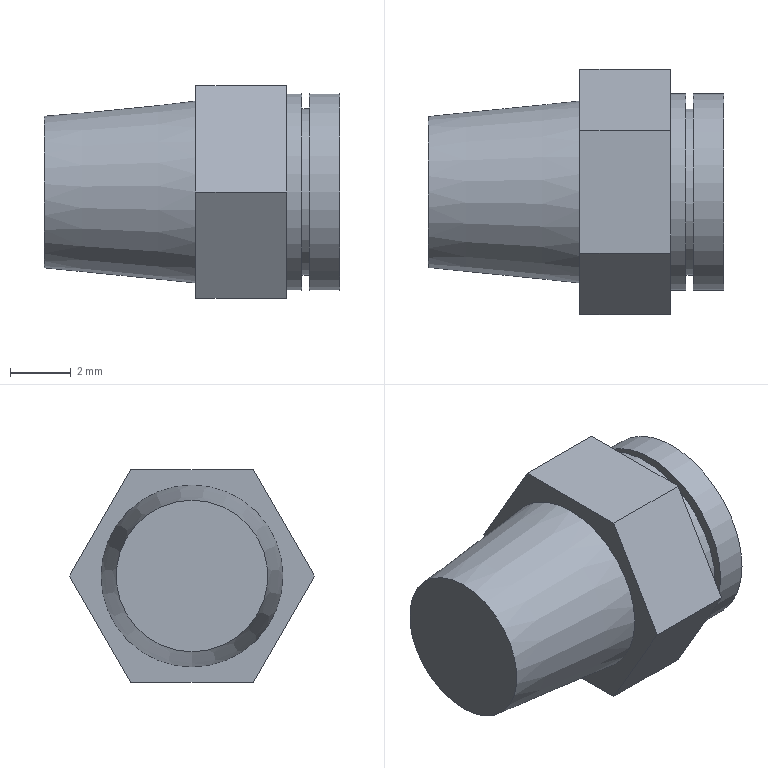Component | NX | AIR_HOSE_CONN_2 | 1 solid | 18 faces | box 9.75 x 8.08 x 7 mm | volume 175 mm3 | plane 13 | cylinder 4 | cone 1 | commonest cylinder face diameters 6.5 x2 5.5 x1 5 x1
STEP:
#1=CARTESIAN_POINT('',(0.,0.,0.));
#2=DIRECTION('',(0.,0.,1.));
#3=DIRECTION('',(1.,0.,0.));
#4=AXIS2_PLACEMENT_3D('',#1,#2,#3);
#5=CARTESIAN_POINT('',(51.,-7.,-6.5));
#6=VERTEX_POINT('',#5);
#7=CARTESIAN_POINT('',(51.,-7.,-4.));
#8=DIRECTION('',(-1.,0.,0.));
#9=DIRECTION('',(0.,0.,-1.));
#10=AXIS2_PLACEMENT_3D('',#7,#8,#9);
#11=CIRCLE('',#10,2.5);
#12=CARTESIAN_POINT('',(56.,-7.,-4.));
#13=DIRECTION('',(1.,0.,0.));
#14=DIRECTION('',(0.,0.,1.));
#15=AXIS2_PLACEMENT_3D('',#12,#13,#14);
#16=CONICAL_SURFACE('',#15,3.,0.09967);
#17=CARTESIAN_POINT('',(9.425,-5.));
#18=DIRECTION('',(-1.,0.));
#19=VECTOR('',#18,1.);
#20=LINE('',#17,#19);
#21=(GEOMETRIC_REPRESENTATION_CONTEXT(2)PARAMETRIC_REPRESENTATION_CONTEXT()REPRESENTATION_CONTEXT('',''));
#22=DEFINITIONAL_REPRESENTATION('',(#20),#21);
#23=PCURVE('',#16,#22);
#24=CARTESIAN_POINT('',(51.,-7.,-1.5));
#25=DIRECTION('',(1.,0.,0.));
#26=DIRECTION('',(0.,0.,1.));
#27=AXIS2_PLACEMENT_3D('',#24,#25,#26);
#28=PLANE('',#27);
#29=CARTESIAN_POINT('',(-5.,0.));
#30=CARTESIAN_POINT('',(-5.,4.33));
#31=CARTESIAN_POINT('',(-1.25,2.165));
#32=CARTESIAN_POINT('',(2.5,0.));
#33=CARTESIAN_POINT('',(-1.25,-2.165));
#34=CARTESIAN_POINT('',(-5.,-4.33));
#35=CARTESIAN_POINT('',(-5.,0.));
#36=(BOUNDED_CURVE()B_SPLINE_CURVE(2,(#29,#30,#31,#32,#33,#34,#35),.UNSPECIFIED.,.T.,.F.)B_SPLINE_CURVE_WITH_KNOTS((1,2,2,2,2,1),(-2.094,0.,2.094,4.189,6.283,8.378),.UNSPECIFIED.)CURVE()GEOMETRIC_REPRESENTATION_ITEM()RATIONAL_B_SPLINE_CURVE((1.,0.5,1.,0.5,1.,0.5,1.))REPRESENTATION_ITEM(''));
#37=(GEOMETRIC_REPRESENTATION_CONTEXT(2)PARAMETRIC_REPRESENTATION_CONTEXT()REPRESENTATION_CONTEXT('',''));
#38=DEFINITIONAL_REPRESENTATION('',(#36),#37);
#39=PCURVE('',#28,#38);
#40=SURFACE_CURVE('',#11,(#23,#39),.PCURVE_S1.);
#41=EDGE_CURVE('',#6,#6,#40,.T.);
#42=ORIENTED_EDGE('',*,*,#41,.F.);
#43=CARTESIAN_POINT('',(56.,-7.,-7.));
#44=VERTEX_POINT('',#43);
#45=CARTESIAN_POINT('',(51.,-7.,-6.5));
#46=CARTESIAN_POINT('',(56.,-7.,-7.));
#47=B_SPLINE_CURVE_WITH_KNOTS('',1,(#45,#46),.UNSPECIFIED.,.F.,.F.,(2,2),(-5.025,0.),.PIECEWISE_BEZIER_KNOTS.);
#48=CARTESIAN_POINT('',(9.425,0.));
#49=DIRECTION('',(0.,1.));
#50=VECTOR('',#49,1.);
#51=LINE('',#48,#50);
#52=(GEOMETRIC_REPRESENTATION_CONTEXT(2)PARAMETRIC_REPRESENTATION_CONTEXT()REPRESENTATION_CONTEXT('',''));
#53=DEFINITIONAL_REPRESENTATION('',(#51),#52);
#54=PCURVE('',#16,#53);
#55=CARTESIAN_POINT('',(3.142,0.));
#56=DIRECTION('',(0.,1.));
#57=VECTOR('',#56,1.);
#58=LINE('',#55,#57);
#59=(GEOMETRIC_REPRESENTATION_CONTEXT(2)PARAMETRIC_REPRESENTATION_CONTEXT()REPRESENTATION_CONTEXT('',''));
#60=DEFINITIONAL_REPRESENTATION('',(#58),#59);
#61=PCURVE('',#16,#60);
#62=SEAM_CURVE('',#47,(#54,#61),.PCURVE_S1.);
#63=EDGE_CURVE('',#6,#44,#62,.T.);
#64=ORIENTED_EDGE('',*,*,#63,.T.);
#65=CARTESIAN_POINT('',(56.,-7.,-4.));
#66=DIRECTION('',(-1.,0.,0.));
#67=DIRECTION('',(0.,0.,-1.));
#68=AXIS2_PLACEMENT_3D('',#65,#66,#67);
#69=CIRCLE('',#68,3.);
#70=CARTESIAN_POINT('',(9.425,0.));
#71=DIRECTION('',(-1.,0.));
#72=VECTOR('',#71,1.);
#73=LINE('',#70,#72);
#74=(GEOMETRIC_REPRESENTATION_CONTEXT(2)PARAMETRIC_REPRESENTATION_CONTEXT()REPRESENTATION_CONTEXT('',''));
#75=DEFINITIONAL_REPRESENTATION('',(#73),#74);
#76=PCURVE('',#16,#75);
#77=CARTESIAN_POINT('',(56.,-7.,-4.));
#78=DIRECTION('',(-1.,0.,0.));
#79=DIRECTION('',(0.,0.,-1.));
#80=AXIS2_PLACEMENT_3D('',#77,#78,#79);
#81=PLANE('',#80);
#82=CARTESIAN_POINT('',(0.,0.));
#83=DIRECTION('',(1.,0.));
#84=AXIS2_PLACEMENT_2D('',#82,#83);
#85=CIRCLE('',#84,3.);
#86=(GEOMETRIC_REPRESENTATION_CONTEXT(2)PARAMETRIC_REPRESENTATION_CONTEXT()REPRESENTATION_CONTEXT('',''));
#87=DEFINITIONAL_REPRESENTATION('',(#85),#86);
#88=PCURVE('',#81,#87);
#89=SURFACE_CURVE('',#69,(#76,#88),.PCURVE_S1.);
#90=EDGE_CURVE('',#44,#44,#89,.T.);
#91=ORIENTED_EDGE('',*,*,#90,.T.);
#92=ORIENTED_EDGE('',*,*,#63,.F.);
#93=EDGE_LOOP('',(#42,#64,#91,#92));
#94=FACE_BOUND('',#93,.T.);
#95=ADVANCED_FACE('',(#94),#16,.T.);
#96=ORIENTED_EDGE('',*,*,#41,.T.);
#97=EDGE_LOOP('',(#96));
#98=FACE_BOUND('',#97,.T.);
#99=ADVANCED_FACE('',(#98),#28,.F.);
#100=CARTESIAN_POINT('',(56.,-4.979,-7.5));
#101=VERTEX_POINT('',#100);
#102=CARTESIAN_POINT('',(56.,-9.021,-7.5));
#103=VERTEX_POINT('',#102);
#104=CARTESIAN_POINT('',(56.,-4.979,-7.5));
#105=DIRECTION('',(0.,-1.,0.));
#106=VECTOR('',#105,1.);
#107=LINE('',#104,#106);
#108=CARTESIAN_POINT('',(59.,-4.979,-7.5));
#109=DIRECTION('',(0.,-0.,-1.));
#110=DIRECTION('',(0.,1.,-0.));
#111=AXIS2_PLACEMENT_3D('',#108,#109,#110);
#112=PLANE('',#111);
#113=CARTESIAN_POINT('',(0.,-3.));
#114=DIRECTION('',(-1.,0.));
#115=VECTOR('',#114,1.);
#116=LINE('',#113,#115);
#117=(GEOMETRIC_REPRESENTATION_CONTEXT(2)PARAMETRIC_REPRESENTATION_CONTEXT()REPRESENTATION_CONTEXT('',''));
#118=DEFINITIONAL_REPRESENTATION('',(#116),#117);
#119=PCURVE('',#112,#118);
#120=CARTESIAN_POINT('',(3.5,-2.021));
#121=DIRECTION('',(-0.,1.));
#122=VECTOR('',#121,1.);
#123=LINE('',#120,#122);
#124=(GEOMETRIC_REPRESENTATION_CONTEXT(2)PARAMETRIC_REPRESENTATION_CONTEXT()REPRESENTATION_CONTEXT('',''));
#125=DEFINITIONAL_REPRESENTATION('',(#123),#124);
#126=PCURVE('',#81,#125);
#127=SURFACE_CURVE('',#107,(#119,#126),.PCURVE_S1.);
#128=EDGE_CURVE('',#101,#103,#127,.T.);
#129=ORIENTED_EDGE('',*,*,#128,.F.);
#130=CARTESIAN_POINT('',(59.,-4.979,-7.5));
#131=VERTEX_POINT('',#130);
#132=CARTESIAN_POINT('',(59.,-4.979,-7.5));
#133=DIRECTION('',(-1.,0.,0.));
#134=VECTOR('',#133,1.);
#135=LINE('',#132,#134);
#136=CARTESIAN_POINT('',(0.,0.));
#137=DIRECTION('',(0.,-1.));
#138=VECTOR('',#137,1.);
#139=LINE('',#136,#138);
#140=(GEOMETRIC_REPRESENTATION_CONTEXT(2)PARAMETRIC_REPRESENTATION_CONTEXT()REPRESENTATION_CONTEXT('',''));
#141=DEFINITIONAL_REPRESENTATION('',(#139),#140);
#142=PCURVE('',#112,#141);
#143=CARTESIAN_POINT('',(59.,-2.959,-4.));
#144=DIRECTION('',(0.,0.866,-0.5));
#145=DIRECTION('',(0.,0.5,0.866));
#146=AXIS2_PLACEMENT_3D('',#143,#144,#145);
#147=PLANE('',#146);
#148=CARTESIAN_POINT('',(-4.041,0.));
#149=DIRECTION('',(0.,-1.));
#150=VECTOR('',#149,1.);
#151=LINE('',#148,#150);
#152=(GEOMETRIC_REPRESENTATION_CONTEXT(2)PARAMETRIC_REPRESENTATION_CONTEXT()REPRESENTATION_CONTEXT('',''));
#153=DEFINITIONAL_REPRESENTATION('',(#151),#152);
#154=PCURVE('',#147,#153);
#155=SURFACE_CURVE('',#135,(#142,#154),.PCURVE_S1.);
#156=EDGE_CURVE('',#131,#101,#155,.T.);
#157=ORIENTED_EDGE('',*,*,#156,.F.);
#158=CARTESIAN_POINT('',(59.,-9.021,-7.5));
#159=VERTEX_POINT('',#158);
#160=CARTESIAN_POINT('',(59.,-4.979,-7.5));
#161=DIRECTION('',(0.,-1.,0.));
#162=VECTOR('',#161,1.);
#163=LINE('',#160,#162);
#164=CARTESIAN_POINT('',(0.,0.));
#165=DIRECTION('',(-1.,0.));
#166=VECTOR('',#165,1.);
#167=LINE('',#164,#166);
#168=(GEOMETRIC_REPRESENTATION_CONTEXT(2)PARAMETRIC_REPRESENTATION_CONTEXT()REPRESENTATION_CONTEXT('',''));
#169=DEFINITIONAL_REPRESENTATION('',(#167),#168);
#170=PCURVE('',#112,#169);
#171=CARTESIAN_POINT('',(59.,-7.,-4.));
#172=DIRECTION('',(-1.,0.,0.));
#173=DIRECTION('',(0.,0.,-1.));
#174=AXIS2_PLACEMENT_3D('',#171,#172,#173);
#175=PLANE('',#174);
#176=CARTESIAN_POINT('',(3.5,-2.021));
#177=DIRECTION('',(-0.,1.));
#178=VECTOR('',#177,1.);
#179=LINE('',#176,#178);
#180=(GEOMETRIC_REPRESENTATION_CONTEXT(2)PARAMETRIC_REPRESENTATION_CONTEXT()REPRESENTATION_CONTEXT('',''));
#181=DEFINITIONAL_REPRESENTATION('',(#179),#180);
#182=PCURVE('',#175,#181);
#183=SURFACE_CURVE('',#163,(#170,#182),.PCURVE_S1.);
#184=EDGE_CURVE('',#131,#159,#183,.T.);
#185=ORIENTED_EDGE('',*,*,#184,.T.);
#186=CARTESIAN_POINT('',(59.,-9.021,-7.5));
#187=DIRECTION('',(-1.,0.,0.));
#188=VECTOR('',#187,1.);
#189=LINE('',#186,#188);
#190=CARTESIAN_POINT('',(-4.041,0.));
#191=DIRECTION('',(0.,-1.));
#192=VECTOR('',#191,1.);
#193=LINE('',#190,#192);
#194=(GEOMETRIC_REPRESENTATION_CONTEXT(2)PARAMETRIC_REPRESENTATION_CONTEXT()REPRESENTATION_CONTEXT('',''));
#195=DEFINITIONAL_REPRESENTATION('',(#193),#194);
#196=PCURVE('',#112,#195);
#197=CARTESIAN_POINT('',(59.,-9.021,-7.5));
#198=DIRECTION('',(0.,-0.866,-0.5));
#199=DIRECTION('',(0.,0.5,-0.866));
#200=AXIS2_PLACEMENT_3D('',#197,#198,#199);
#201=PLANE('',#200);
#202=CARTESIAN_POINT('',(0.,0.));
#203=DIRECTION('',(0.,-1.));
#204=VECTOR('',#203,1.);
#205=LINE('',#202,#204);
#206=(GEOMETRIC_REPRESENTATION_CONTEXT(2)PARAMETRIC_REPRESENTATION_CONTEXT()REPRESENTATION_CONTEXT('',''));
#207=DEFINITIONAL_REPRESENTATION('',(#205),#206);
#208=PCURVE('',#201,#207);
#209=SURFACE_CURVE('',#189,(#196,#208),.PCURVE_S1.);
#210=EDGE_CURVE('',#159,#103,#209,.T.);
#211=ORIENTED_EDGE('',*,*,#210,.T.);
#212=EDGE_LOOP('',(#129,#157,#185,#211));
#213=FACE_BOUND('',#212,.T.);
#214=ADVANCED_FACE('',(#213),#112,.T.);
#215=CARTESIAN_POINT('',(56.,-11.041,-4.));
#216=VERTEX_POINT('',#215);
#217=CARTESIAN_POINT('',(56.,-9.021,-7.5));
#218=DIRECTION('',(0.,-0.5,0.866));
#219=VECTOR('',#218,1.);
#220=LINE('',#217,#219);
#221=CARTESIAN_POINT('',(0.,-3.));
#222=DIRECTION('',(-1.,0.));
#223=VECTOR('',#222,1.);
#224=LINE('',#221,#223);
#225=(GEOMETRIC_REPRESENTATION_CONTEXT(2)PARAMETRIC_REPRESENTATION_CONTEXT()REPRESENTATION_CONTEXT('',''));
#226=DEFINITIONAL_REPRESENTATION('',(#224),#225);
#227=PCURVE('',#201,#226);
#228=CARTESIAN_POINT('',(3.5,2.021));
#229=DIRECTION('',(-0.866,0.5));
#230=VECTOR('',#229,1.);
#231=LINE('',#228,#230);
#232=(GEOMETRIC_REPRESENTATION_CONTEXT(2)PARAMETRIC_REPRESENTATION_CONTEXT()REPRESENTATION_CONTEXT('',''));
#233=DEFINITIONAL_REPRESENTATION('',(#231),#232);
#234=PCURVE('',#81,#233);
#235=SURFACE_CURVE('',#220,(#227,#234),.PCURVE_S1.);
#236=EDGE_CURVE('',#103,#216,#235,.T.);
#237=ORIENTED_EDGE('',*,*,#236,.F.);
#238=ORIENTED_EDGE('',*,*,#210,.F.);
#239=CARTESIAN_POINT('',(59.,-11.041,-4.));
#240=VERTEX_POINT('',#239);
#241=CARTESIAN_POINT('',(59.,-9.021,-7.5));
#242=DIRECTION('',(0.,-0.5,0.866));
#243=VECTOR('',#242,1.);
#244=LINE('',#241,#243);
#245=CARTESIAN_POINT('',(0.,0.));
#246=DIRECTION('',(-1.,0.));
#247=VECTOR('',#246,1.);
#248=LINE('',#245,#247);
#249=(GEOMETRIC_REPRESENTATION_CONTEXT(2)PARAMETRIC_REPRESENTATION_CONTEXT()REPRESENTATION_CONTEXT('',''));
#250=DEFINITIONAL_REPRESENTATION('',(#248),#249);
#251=PCURVE('',#201,#250);
#252=CARTESIAN_POINT('',(3.5,2.021));
#253=DIRECTION('',(-0.866,0.5));
#254=VECTOR('',#253,1.);
#255=LINE('',#252,#254);
#256=(GEOMETRIC_REPRESENTATION_CONTEXT(2)PARAMETRIC_REPRESENTATION_CONTEXT()REPRESENTATION_CONTEXT('',''));
#257=DEFINITIONAL_REPRESENTATION('',(#255),#256);
#258=PCURVE('',#175,#257);
#259=SURFACE_CURVE('',#244,(#251,#258),.PCURVE_S1.);
#260=EDGE_CURVE('',#159,#240,#259,.T.);
#261=ORIENTED_EDGE('',*,*,#260,.T.);
#262=CARTESIAN_POINT('',(59.,-11.041,-4.));
#263=DIRECTION('',(-1.,0.,0.));
#264=VECTOR('',#263,1.);
#265=LINE('',#262,#264);
#266=CARTESIAN_POINT('',(-4.041,0.));
#267=DIRECTION('',(0.,-1.));
#268=VECTOR('',#267,1.);
#269=LINE('',#266,#268);
#270=(GEOMETRIC_REPRESENTATION_CONTEXT(2)PARAMETRIC_REPRESENTATION_CONTEXT()REPRESENTATION_CONTEXT('',''));
#271=DEFINITIONAL_REPRESENTATION('',(#269),#270);
#272=PCURVE('',#201,#271);
#273=CARTESIAN_POINT('',(59.,-11.041,-4.));
#274=DIRECTION('',(0.,-0.866,0.5));
#275=DIRECTION('',(0.,-0.5,-0.866));
#276=AXIS2_PLACEMENT_3D('',#273,#274,#275);
#277=PLANE('',#276);
#278=CARTESIAN_POINT('',(0.,0.));
#279=DIRECTION('',(0.,-1.));
#280=VECTOR('',#279,1.);
#281=LINE('',#278,#280);
#282=(GEOMETRIC_REPRESENTATION_CONTEXT(2)PARAMETRIC_REPRESENTATION_CONTEXT()REPRESENTATION_CONTEXT('',''));
#283=DEFINITIONAL_REPRESENTATION('',(#281),#282);
#284=PCURVE('',#277,#283);
#285=SURFACE_CURVE('',#265,(#272,#284),.PCURVE_S1.);
#286=EDGE_CURVE('',#240,#216,#285,.T.);
#287=ORIENTED_EDGE('',*,*,#286,.T.);
#288=EDGE_LOOP('',(#237,#238,#261,#287));
#289=FACE_BOUND('',#288,.T.);
#290=ADVANCED_FACE('',(#289),#201,.T.);
#291=CARTESIAN_POINT('',(56.,-9.021,-0.5));
#292=VERTEX_POINT('',#291);
#293=CARTESIAN_POINT('',(56.,-11.041,-4.));
#294=DIRECTION('',(0.,0.5,0.866));
#295=VECTOR('',#294,1.);
#296=LINE('',#293,#295);
#297=CARTESIAN_POINT('',(0.,-3.));
#298=DIRECTION('',(-1.,0.));
#299=VECTOR('',#298,1.);
#300=LINE('',#297,#299);
#301=(GEOMETRIC_REPRESENTATION_CONTEXT(2)PARAMETRIC_REPRESENTATION_CONTEXT()REPRESENTATION_CONTEXT('',''));
#302=DEFINITIONAL_REPRESENTATION('',(#300),#301);
#303=PCURVE('',#277,#302);
#304=CARTESIAN_POINT('',(-0.,4.041));
#305=DIRECTION('',(-0.866,-0.5));
#306=VECTOR('',#305,1.);
#307=LINE('',#304,#306);
#308=(GEOMETRIC_REPRESENTATION_CONTEXT(2)PARAMETRIC_REPRESENTATION_CONTEXT()REPRESENTATION_CONTEXT('',''));
#309=DEFINITIONAL_REPRESENTATION('',(#307),#308);
#310=PCURVE('',#81,#309);
#311=SURFACE_CURVE('',#296,(#303,#310),.PCURVE_S1.);
#312=EDGE_CURVE('',#216,#292,#311,.T.);
#313=ORIENTED_EDGE('',*,*,#312,.F.);
#314=ORIENTED_EDGE('',*,*,#286,.F.);
#315=CARTESIAN_POINT('',(59.,-9.021,-0.5));
#316=VERTEX_POINT('',#315);
#317=CARTESIAN_POINT('',(59.,-11.041,-4.));
#318=DIRECTION('',(0.,0.5,0.866));
#319=VECTOR('',#318,1.);
#320=LINE('',#317,#319);
#321=CARTESIAN_POINT('',(0.,0.));
#322=DIRECTION('',(-1.,0.));
#323=VECTOR('',#322,1.);
#324=LINE('',#321,#323);
#325=(GEOMETRIC_REPRESENTATION_CONTEXT(2)PARAMETRIC_REPRESENTATION_CONTEXT()REPRESENTATION_CONTEXT('',''));
#326=DEFINITIONAL_REPRESENTATION('',(#324),#325);
#327=PCURVE('',#277,#326);
#328=CARTESIAN_POINT('',(-0.,4.041));
#329=DIRECTION('',(-0.866,-0.5));
#330=VECTOR('',#329,1.);
#331=LINE('',#328,#330);
#332=(GEOMETRIC_REPRESENTATION_CONTEXT(2)PARAMETRIC_REPRESENTATION_CONTEXT()REPRESENTATION_CONTEXT('',''));
#333=DEFINITIONAL_REPRESENTATION('',(#331),#332);
#334=PCURVE('',#175,#333);
#335=SURFACE_CURVE('',#320,(#327,#334),.PCURVE_S1.);
#336=EDGE_CURVE('',#240,#316,#335,.T.);
#337=ORIENTED_EDGE('',*,*,#336,.T.);
#338=CARTESIAN_POINT('',(59.,-9.021,-0.5));
#339=DIRECTION('',(-1.,0.,0.));
#340=VECTOR('',#339,1.);
#341=LINE('',#338,#340);
#342=CARTESIAN_POINT('',(-4.041,0.));
#343=DIRECTION('',(0.,-1.));
#344=VECTOR('',#343,1.);
#345=LINE('',#342,#344);
#346=(GEOMETRIC_REPRESENTATION_CONTEXT(2)PARAMETRIC_REPRESENTATION_CONTEXT()REPRESENTATION_CONTEXT('',''));
#347=DEFINITIONAL_REPRESENTATION('',(#345),#346);
#348=PCURVE('',#277,#347);
#349=CARTESIAN_POINT('',(59.,-9.021,-0.5));
#350=DIRECTION('',(0.,0.,1.));
#351=DIRECTION('',(0.,-1.,0.));
#352=AXIS2_PLACEMENT_3D('',#349,#350,#351);
#353=PLANE('',#352);
#354=CARTESIAN_POINT('',(0.,0.));
#355=DIRECTION('',(0.,-1.));
#356=VECTOR('',#355,1.);
#357=LINE('',#354,#356);
#358=(GEOMETRIC_REPRESENTATION_CONTEXT(2)PARAMETRIC_REPRESENTATION_CONTEXT()REPRESENTATION_CONTEXT('',''));
#359=DEFINITIONAL_REPRESENTATION('',(#357),#358);
#360=PCURVE('',#353,#359);
#361=SURFACE_CURVE('',#341,(#348,#360),.PCURVE_S1.);
#362=EDGE_CURVE('',#316,#292,#361,.T.);
#363=ORIENTED_EDGE('',*,*,#362,.T.);
#364=EDGE_LOOP('',(#313,#314,#337,#363));
#365=FACE_BOUND('',#364,.T.);
#366=ADVANCED_FACE('',(#365),#277,.T.);
#367=CARTESIAN_POINT('',(56.,-4.979,-0.5));
#368=VERTEX_POINT('',#367);
#369=CARTESIAN_POINT('',(56.,-9.021,-0.5));
#370=DIRECTION('',(0.,1.,-0.));
#371=VECTOR('',#370,1.);
#372=LINE('',#369,#371);
#373=CARTESIAN_POINT('',(0.,-3.));
#374=DIRECTION('',(-1.,0.));
#375=VECTOR('',#374,1.);
#376=LINE('',#373,#375);
#377=(GEOMETRIC_REPRESENTATION_CONTEXT(2)PARAMETRIC_REPRESENTATION_CONTEXT()REPRESENTATION_CONTEXT('',''));
#378=DEFINITIONAL_REPRESENTATION('',(#376),#377);
#379=PCURVE('',#353,#378);
#380=CARTESIAN_POINT('',(-3.5,2.021));
#381=DIRECTION('',(0.,-1.));
#382=VECTOR('',#381,1.);
#383=LINE('',#380,#382);
#384=(GEOMETRIC_REPRESENTATION_CONTEXT(2)PARAMETRIC_REPRESENTATION_CONTEXT()REPRESENTATION_CONTEXT('',''));
#385=DEFINITIONAL_REPRESENTATION('',(#383),#384);
#386=PCURVE('',#81,#385);
#387=SURFACE_CURVE('',#372,(#379,#386),.PCURVE_S1.);
#388=EDGE_CURVE('',#292,#368,#387,.T.);
#389=ORIENTED_EDGE('',*,*,#388,.F.);
#390=ORIENTED_EDGE('',*,*,#362,.F.);
#391=CARTESIAN_POINT('',(59.,-4.979,-0.5));
#392=VERTEX_POINT('',#391);
#393=CARTESIAN_POINT('',(59.,-9.021,-0.5));
#394=DIRECTION('',(0.,1.,-0.));
#395=VECTOR('',#394,1.);
#396=LINE('',#393,#395);
#397=CARTESIAN_POINT('',(0.,0.));
#398=DIRECTION('',(-1.,0.));
#399=VECTOR('',#398,1.);
#400=LINE('',#397,#399);
#401=(GEOMETRIC_REPRESENTATION_CONTEXT(2)PARAMETRIC_REPRESENTATION_CONTEXT()REPRESENTATION_CONTEXT('',''));
#402=DEFINITIONAL_REPRESENTATION('',(#400),#401);
#403=PCURVE('',#353,#402);
#404=CARTESIAN_POINT('',(-3.5,2.021));
#405=DIRECTION('',(0.,-1.));
#406=VECTOR('',#405,1.);
#407=LINE('',#404,#406);
#408=(GEOMETRIC_REPRESENTATION_CONTEXT(2)PARAMETRIC_REPRESENTATION_CONTEXT()REPRESENTATION_CONTEXT('',''));
#409=DEFINITIONAL_REPRESENTATION('',(#407),#408);
#410=PCURVE('',#175,#409);
#411=SURFACE_CURVE('',#396,(#403,#410),.PCURVE_S1.);
#412=EDGE_CURVE('',#316,#392,#411,.T.);
#413=ORIENTED_EDGE('',*,*,#412,.T.);
#414=CARTESIAN_POINT('',(59.,-4.979,-0.5));
#415=DIRECTION('',(-1.,0.,0.));
#416=VECTOR('',#415,1.);
#417=LINE('',#414,#416);
#418=CARTESIAN_POINT('',(-4.041,0.));
#419=DIRECTION('',(0.,-1.));
#420=VECTOR('',#419,1.);
#421=LINE('',#418,#420);
#422=(GEOMETRIC_REPRESENTATION_CONTEXT(2)PARAMETRIC_REPRESENTATION_CONTEXT()REPRESENTATION_CONTEXT('',''));
#423=DEFINITIONAL_REPRESENTATION('',(#421),#422);
#424=PCURVE('',#353,#423);
#425=CARTESIAN_POINT('',(59.,-4.979,-0.5));
#426=DIRECTION('',(0.,0.866,0.5));
#427=DIRECTION('',(0.,-0.5,0.866));
#428=AXIS2_PLACEMENT_3D('',#425,#426,#427);
#429=PLANE('',#428);
#430=CARTESIAN_POINT('',(0.,0.));
#431=DIRECTION('',(0.,-1.));
#432=VECTOR('',#431,1.);
#433=LINE('',#430,#432);
#434=(GEOMETRIC_REPRESENTATION_CONTEXT(2)PARAMETRIC_REPRESENTATION_CONTEXT()REPRESENTATION_CONTEXT('',''));
#435=DEFINITIONAL_REPRESENTATION('',(#433),#434);
#436=PCURVE('',#429,#435);
#437=SURFACE_CURVE('',#417,(#424,#436),.PCURVE_S1.);
#438=EDGE_CURVE('',#392,#368,#437,.T.);
#439=ORIENTED_EDGE('',*,*,#438,.T.);
#440=EDGE_LOOP('',(#389,#390,#413,#439));
#441=FACE_BOUND('',#440,.T.);
#442=ADVANCED_FACE('',(#441),#353,.T.);
#443=CARTESIAN_POINT('',(56.,-2.959,-4.));
#444=VERTEX_POINT('',#443);
#445=CARTESIAN_POINT('',(56.,-4.979,-0.5));
#446=DIRECTION('',(0.,0.5,-0.866));
#447=VECTOR('',#446,1.);
#448=LINE('',#445,#447);
#449=CARTESIAN_POINT('',(0.,-3.));
#450=DIRECTION('',(-1.,0.));
#451=VECTOR('',#450,1.);
#452=LINE('',#449,#451);
#453=(GEOMETRIC_REPRESENTATION_CONTEXT(2)PARAMETRIC_REPRESENTATION_CONTEXT()REPRESENTATION_CONTEXT('',''));
#454=DEFINITIONAL_REPRESENTATION('',(#452),#453);
#455=PCURVE('',#429,#454);
#456=CARTESIAN_POINT('',(-3.5,-2.021));
#457=DIRECTION('',(0.866,-0.5));
#458=VECTOR('',#457,1.);
#459=LINE('',#456,#458);
#460=(GEOMETRIC_REPRESENTATION_CONTEXT(2)PARAMETRIC_REPRESENTATION_CONTEXT()REPRESENTATION_CONTEXT('',''));
#461=DEFINITIONAL_REPRESENTATION('',(#459),#460);
#462=PCURVE('',#81,#461);
#463=SURFACE_CURVE('',#448,(#455,#462),.PCURVE_S1.);
#464=EDGE_CURVE('',#368,#444,#463,.T.);
#465=ORIENTED_EDGE('',*,*,#464,.F.);
#466=ORIENTED_EDGE('',*,*,#438,.F.);
#467=CARTESIAN_POINT('',(59.,-2.959,-4.));
#468=VERTEX_POINT('',#467);
#469=CARTESIAN_POINT('',(59.,-4.979,-0.5));
#470=DIRECTION('',(0.,0.5,-0.866));
#471=VECTOR('',#470,1.);
#472=LINE('',#469,#471);
#473=CARTESIAN_POINT('',(0.,0.));
#474=DIRECTION('',(-1.,0.));
#475=VECTOR('',#474,1.);
#476=LINE('',#473,#475);
#477=(GEOMETRIC_REPRESENTATION_CONTEXT(2)PARAMETRIC_REPRESENTATION_CONTEXT()REPRESENTATION_CONTEXT('',''));
#478=DEFINITIONAL_REPRESENTATION('',(#476),#477);
#479=PCURVE('',#429,#478);
#480=CARTESIAN_POINT('',(-3.5,-2.021));
#481=DIRECTION('',(0.866,-0.5));
#482=VECTOR('',#481,1.);
#483=LINE('',#480,#482);
#484=(GEOMETRIC_REPRESENTATION_CONTEXT(2)PARAMETRIC_REPRESENTATION_CONTEXT()REPRESENTATION_CONTEXT('',''));
#485=DEFINITIONAL_REPRESENTATION('',(#483),#484);
#486=PCURVE('',#175,#485);
#487=SURFACE_CURVE('',#472,(#479,#486),.PCURVE_S1.);
#488=EDGE_CURVE('',#392,#468,#487,.T.);
#489=ORIENTED_EDGE('',*,*,#488,.T.);
#490=CARTESIAN_POINT('',(59.,-2.959,-4.));
#491=DIRECTION('',(-1.,0.,0.));
#492=VECTOR('',#491,1.);
#493=LINE('',#490,#492);
#494=CARTESIAN_POINT('',(-4.041,0.));
#495=DIRECTION('',(0.,-1.));
#496=VECTOR('',#495,1.);
#497=LINE('',#494,#496);
#498=(GEOMETRIC_REPRESENTATION_CONTEXT(2)PARAMETRIC_REPRESENTATION_CONTEXT()REPRESENTATION_CONTEXT('',''));
#499=DEFINITIONAL_REPRESENTATION('',(#497),#498);
#500=PCURVE('',#429,#499);
#501=CARTESIAN_POINT('',(0.,0.));
#502=DIRECTION('',(0.,-1.));
#503=VECTOR('',#502,1.);
#504=LINE('',#501,#503);
#505=(GEOMETRIC_REPRESENTATION_CONTEXT(2)PARAMETRIC_REPRESENTATION_CONTEXT()REPRESENTATION_CONTEXT('',''));
#506=DEFINITIONAL_REPRESENTATION('',(#504),#505);
#507=PCURVE('',#147,#506);
#508=SURFACE_CURVE('',#493,(#500,#507),.PCURVE_S1.);
#509=EDGE_CURVE('',#468,#444,#508,.T.);
#510=ORIENTED_EDGE('',*,*,#509,.T.);
#511=EDGE_LOOP('',(#465,#466,#489,#510));
#512=FACE_BOUND('',#511,.T.);
#513=ADVANCED_FACE('',(#512),#429,.T.);
#514=CARTESIAN_POINT('',(56.,-2.959,-4.));
#515=DIRECTION('',(0.,-0.5,-0.866));
#516=VECTOR('',#515,1.);
#517=LINE('',#514,#516);
#518=CARTESIAN_POINT('',(0.,-3.));
#519=DIRECTION('',(-1.,0.));
#520=VECTOR('',#519,1.);
#521=LINE('',#518,#520);
#522=(GEOMETRIC_REPRESENTATION_CONTEXT(2)PARAMETRIC_REPRESENTATION_CONTEXT()REPRESENTATION_CONTEXT('',''));
#523=DEFINITIONAL_REPRESENTATION('',(#521),#522);
#524=PCURVE('',#147,#523);
#525=CARTESIAN_POINT('',(0.,-4.041));
#526=DIRECTION('',(0.866,0.5));
#527=VECTOR('',#526,1.);
#528=LINE('',#525,#527);
#529=(GEOMETRIC_REPRESENTATION_CONTEXT(2)PARAMETRIC_REPRESENTATION_CONTEXT()REPRESENTATION_CONTEXT('',''));
#530=DEFINITIONAL_REPRESENTATION('',(#528),#529);
#531=PCURVE('',#81,#530);
#532=SURFACE_CURVE('',#517,(#524,#531),.PCURVE_S1.);
#533=EDGE_CURVE('',#444,#101,#532,.T.);
#534=ORIENTED_EDGE('',*,*,#533,.F.);
#535=ORIENTED_EDGE('',*,*,#509,.F.);
#536=CARTESIAN_POINT('',(59.,-2.959,-4.));
#537=DIRECTION('',(0.,-0.5,-0.866));
#538=VECTOR('',#537,1.);
#539=LINE('',#536,#538);
#540=CARTESIAN_POINT('',(0.,0.));
#541=DIRECTION('',(-1.,0.));
#542=VECTOR('',#541,1.);
#543=LINE('',#540,#542);
#544=(GEOMETRIC_REPRESENTATION_CONTEXT(2)PARAMETRIC_REPRESENTATION_CONTEXT()REPRESENTATION_CONTEXT('',''));
#545=DEFINITIONAL_REPRESENTATION('',(#543),#544);
#546=PCURVE('',#147,#545);
#547=CARTESIAN_POINT('',(0.,-4.041));
#548=DIRECTION('',(0.866,0.5));
#549=VECTOR('',#548,1.);
#550=LINE('',#547,#549);
#551=(GEOMETRIC_REPRESENTATION_CONTEXT(2)PARAMETRIC_REPRESENTATION_CONTEXT()REPRESENTATION_CONTEXT('',''));
#552=DEFINITIONAL_REPRESENTATION('',(#550),#551);
#553=PCURVE('',#175,#552);
#554=SURFACE_CURVE('',#539,(#546,#553),.PCURVE_S1.);
#555=EDGE_CURVE('',#468,#131,#554,.T.);
#556=ORIENTED_EDGE('',*,*,#555,.T.);
#557=ORIENTED_EDGE('',*,*,#156,.T.);
#558=EDGE_LOOP('',(#534,#535,#556,#557));
#559=FACE_BOUND('',#558,.T.);
#560=ADVANCED_FACE('',(#559),#147,.T.);
#561=CARTESIAN_POINT('',(59.,-3.75,-4.));
#562=VERTEX_POINT('',#561);
#563=CARTESIAN_POINT('',(59.,-7.,-4.));
#564=DIRECTION('',(-1.,0.,0.));
#565=DIRECTION('',(0.,1.,0.));
#566=AXIS2_PLACEMENT_3D('',#563,#564,#565);
#567=CIRCLE('',#566,3.25);
#568=CARTESIAN_POINT('',(0.,0.));
#569=DIRECTION('',(-0.,-1.));
#570=AXIS2_PLACEMENT_2D('',#568,#569);
#571=CIRCLE('',#570,3.25);
#572=(GEOMETRIC_REPRESENTATION_CONTEXT(2)PARAMETRIC_REPRESENTATION_CONTEXT()REPRESENTATION_CONTEXT('',''));
#573=DEFINITIONAL_REPRESENTATION('',(#571),#572);
#574=PCURVE('',#175,#573);
#575=CARTESIAN_POINT('',(59.5,-7.,-4.));
#576=DIRECTION('',(-1.,0.,0.));
#577=DIRECTION('',(0.,0.,-1.));
#578=AXIS2_PLACEMENT_3D('',#575,#576,#577);
#579=CYLINDRICAL_SURFACE('',#578,3.25);
#580=CARTESIAN_POINT('',(4.712,0.5));
#581=DIRECTION('',(1.,0.));
#582=VECTOR('',#581,1.);
#583=LINE('',#580,#582);
#584=(GEOMETRIC_REPRESENTATION_CONTEXT(2)PARAMETRIC_REPRESENTATION_CONTEXT()REPRESENTATION_CONTEXT('',''));
#585=DEFINITIONAL_REPRESENTATION('',(#583),#584);
#586=PCURVE('',#579,#585);
#587=SURFACE_CURVE('',#567,(#574,#586),.PCURVE_S1.);
#588=EDGE_CURVE('',#562,#562,#587,.T.);
#589=ORIENTED_EDGE('',*,*,#588,.T.);
#590=EDGE_LOOP('',(#589));
#591=FACE_BOUND('',#590,.T.);
#592=ORIENTED_EDGE('',*,*,#184,.F.);
#593=ORIENTED_EDGE('',*,*,#555,.F.);
#594=ORIENTED_EDGE('',*,*,#488,.F.);
#595=ORIENTED_EDGE('',*,*,#412,.F.);
#596=ORIENTED_EDGE('',*,*,#336,.F.);
#597=ORIENTED_EDGE('',*,*,#260,.F.);
#598=EDGE_LOOP('',(#592,#593,#594,#595,#596,#597));
#599=FACE_BOUND('',#598,.T.);
#600=ADVANCED_FACE('',(#591,#599),#175,.F.);
#601=ORIENTED_EDGE('',*,*,#90,.F.);
#602=EDGE_LOOP('',(#601));
#603=FACE_BOUND('',#602,.T.);
#604=ORIENTED_EDGE('',*,*,#128,.T.);
#605=ORIENTED_EDGE('',*,*,#236,.T.);
#606=ORIENTED_EDGE('',*,*,#312,.T.);
#607=ORIENTED_EDGE('',*,*,#388,.T.);
#608=ORIENTED_EDGE('',*,*,#464,.T.);
#609=ORIENTED_EDGE('',*,*,#533,.T.);
#610=EDGE_LOOP('',(#604,#605,#606,#607,#608,#609));
#611=FACE_BOUND('',#610,.T.);
#612=ADVANCED_FACE('',(#603,#611),#81,.T.);
#613=CARTESIAN_POINT('',(59.5,-3.75,-4.));
#614=VERTEX_POINT('',#613);
#615=CARTESIAN_POINT('',(59.5,-7.,-4.));
#616=DIRECTION('',(-1.,0.,0.));
#617=DIRECTION('',(0.,1.,0.));
#618=AXIS2_PLACEMENT_3D('',#615,#616,#617);
#619=CIRCLE('',#618,3.25);
#620=CARTESIAN_POINT('',(4.712,0.));
#621=DIRECTION('',(1.,0.));
#622=VECTOR('',#621,1.);
#623=LINE('',#620,#622);
#624=(GEOMETRIC_REPRESENTATION_CONTEXT(2)PARAMETRIC_REPRESENTATION_CONTEXT()REPRESENTATION_CONTEXT('',''));
#625=DEFINITIONAL_REPRESENTATION('',(#623),#624);
#626=PCURVE('',#579,#625);
#627=CARTESIAN_POINT('',(59.5,-7.,-4.));
#628=DIRECTION('',(-1.,0.,0.));
#629=DIRECTION('',(0.,0.,-1.));
#630=AXIS2_PLACEMENT_3D('',#627,#628,#629);
#631=PLANE('',#630);
#632=CARTESIAN_POINT('',(0.,0.));
#633=DIRECTION('',(-0.,-1.));
#634=AXIS2_PLACEMENT_2D('',#632,#633);
#635=CIRCLE('',#634,3.25);
#636=(GEOMETRIC_REPRESENTATION_CONTEXT(2)PARAMETRIC_REPRESENTATION_CONTEXT()REPRESENTATION_CONTEXT('',''));
#637=DEFINITIONAL_REPRESENTATION('',(#635),#636);
#638=PCURVE('',#631,#637);
#639=SURFACE_CURVE('',#619,(#626,#638),.PCURVE_S1.);
#640=EDGE_CURVE('',#614,#614,#639,.T.);
#641=ORIENTED_EDGE('',*,*,#640,.T.);
#642=CARTESIAN_POINT('',(59.5,-3.75,-4.));
#643=CARTESIAN_POINT('',(59.,-3.75,-4.));
#644=B_SPLINE_CURVE_WITH_KNOTS('',1,(#642,#643),.UNSPECIFIED.,.F.,.F.,(2,2),(0.,0.5),.PIECEWISE_BEZIER_KNOTS.);
#645=CARTESIAN_POINT('',(10.996,0.));
#646=DIRECTION('',(0.,1.));
#647=VECTOR('',#646,1.);
#648=LINE('',#645,#647);
#649=(GEOMETRIC_REPRESENTATION_CONTEXT(2)PARAMETRIC_REPRESENTATION_CONTEXT()REPRESENTATION_CONTEXT('',''));
#650=DEFINITIONAL_REPRESENTATION('',(#648),#649);
#651=PCURVE('',#579,#650);
#652=CARTESIAN_POINT('',(4.712,0.));
#653=DIRECTION('',(0.,1.));
#654=VECTOR('',#653,1.);
#655=LINE('',#652,#654);
#656=(GEOMETRIC_REPRESENTATION_CONTEXT(2)PARAMETRIC_REPRESENTATION_CONTEXT()REPRESENTATION_CONTEXT('',''));
#657=DEFINITIONAL_REPRESENTATION('',(#655),#656);
#658=PCURVE('',#579,#657);
#659=SEAM_CURVE('',#644,(#651,#658),.PCURVE_S1.);
#660=EDGE_CURVE('',#614,#562,#659,.T.);
#661=ORIENTED_EDGE('',*,*,#660,.T.);
#662=ORIENTED_EDGE('',*,*,#588,.F.);
#663=ORIENTED_EDGE('',*,*,#660,.F.);
#664=EDGE_LOOP('',(#641,#661,#662,#663));
#665=FACE_BOUND('',#664,.T.);
#666=ADVANCED_FACE('',(#665),#579,.T.);
#667=CARTESIAN_POINT('',(59.5,-9.75,-4.));
#668=VERTEX_POINT('',#667);
#669=CARTESIAN_POINT('',(59.5,-7.,-4.));
#670=DIRECTION('',(1.,0.,0.));
#671=DIRECTION('',(0.,-1.,0.));
#672=AXIS2_PLACEMENT_3D('',#669,#670,#671);
#673=CIRCLE('',#672,2.75);
#674=CARTESIAN_POINT('',(0.,2.75));
#675=CARTESIAN_POINT('',(4.763,2.75));
#676=CARTESIAN_POINT('',(2.382,-1.375));
#677=CARTESIAN_POINT('',(0.,-5.5));
#678=CARTESIAN_POINT('',(-2.382,-1.375));
#679=CARTESIAN_POINT('',(-4.763,2.75));
#680=CARTESIAN_POINT('',(0.,2.75));
#681=(BOUNDED_CURVE()B_SPLINE_CURVE(2,(#674,#675,#676,#677,#678,#679,#680),.UNSPECIFIED.,.T.,.F.)B_SPLINE_CURVE_WITH_KNOTS((1,2,2,2,2,1),(-2.094,0.,2.094,4.189,6.283,8.378),.UNSPECIFIED.)CURVE()GEOMETRIC_REPRESENTATION_ITEM()RATIONAL_B_SPLINE_CURVE((1.,0.5,1.,0.5,1.,0.5,1.))REPRESENTATION_ITEM(''));
#682=(GEOMETRIC_REPRESENTATION_CONTEXT(2)PARAMETRIC_REPRESENTATION_CONTEXT()REPRESENTATION_CONTEXT('',''));
#683=DEFINITIONAL_REPRESENTATION('',(#681),#682);
#684=PCURVE('',#631,#683);
#685=CARTESIAN_POINT('',(59.75,-7.,-4.));
#686=DIRECTION('',(-1.,0.,0.));
#687=DIRECTION('',(0.,0.,-1.));
#688=AXIS2_PLACEMENT_3D('',#685,#686,#687);
#689=CYLINDRICAL_SURFACE('',#688,2.75);
#690=CARTESIAN_POINT('',(7.854,0.25));
#691=DIRECTION('',(-1.,0.));
#692=VECTOR('',#691,1.);
#693=LINE('',#690,#692);
#694=(GEOMETRIC_REPRESENTATION_CONTEXT(2)PARAMETRIC_REPRESENTATION_CONTEXT()REPRESENTATION_CONTEXT('',''));
#695=DEFINITIONAL_REPRESENTATION('',(#693),#694);
#696=PCURVE('',#689,#695);
#697=SURFACE_CURVE('',#673,(#684,#696),.PCURVE_S1.);
#698=EDGE_CURVE('',#668,#668,#697,.T.);
#699=ORIENTED_EDGE('',*,*,#698,.F.);
#700=EDGE_LOOP('',(#699));
#701=FACE_BOUND('',#700,.T.);
#702=ORIENTED_EDGE('',*,*,#640,.F.);
#703=EDGE_LOOP('',(#702));
#704=FACE_BOUND('',#703,.T.);
#705=ADVANCED_FACE('',(#701,#704),#631,.F.);
#706=CARTESIAN_POINT('',(59.75,-9.75,-4.));
#707=VERTEX_POINT('',#706);
#708=CARTESIAN_POINT('',(59.75,-7.,-4.));
#709=DIRECTION('',(1.,0.,0.));
#710=DIRECTION('',(0.,-1.,0.));
#711=AXIS2_PLACEMENT_3D('',#708,#709,#710);
#712=CIRCLE('',#711,2.75);
#713=CARTESIAN_POINT('',(7.854,0.));
#714=DIRECTION('',(-1.,0.));
#715=VECTOR('',#714,1.);
#716=LINE('',#713,#715);
#717=(GEOMETRIC_REPRESENTATION_CONTEXT(2)PARAMETRIC_REPRESENTATION_CONTEXT()REPRESENTATION_CONTEXT('',''));
#718=DEFINITIONAL_REPRESENTATION('',(#716),#717);
#719=PCURVE('',#689,#718);
#720=CARTESIAN_POINT('',(59.75,-7.,-4.));
#721=DIRECTION('',(1.,0.,0.));
#722=DIRECTION('',(0.,0.,1.));
#723=AXIS2_PLACEMENT_3D('',#720,#721,#722);
#724=PLANE('',#723);
#725=CARTESIAN_POINT('',(0.,0.));
#726=DIRECTION('',(0.,1.));
#727=AXIS2_PLACEMENT_2D('',#725,#726);
#728=CIRCLE('',#727,2.75);
#729=(GEOMETRIC_REPRESENTATION_CONTEXT(2)PARAMETRIC_REPRESENTATION_CONTEXT()REPRESENTATION_CONTEXT('',''));
#730=DEFINITIONAL_REPRESENTATION('',(#728),#729);
#731=PCURVE('',#724,#730);
#732=SURFACE_CURVE('',#712,(#719,#731),.PCURVE_S1.);
#733=EDGE_CURVE('',#707,#707,#732,.T.);
#734=ORIENTED_EDGE('',*,*,#733,.F.);
#735=CARTESIAN_POINT('',(59.75,-9.75,-4.));
#736=CARTESIAN_POINT('',(59.5,-9.75,-4.));
#737=B_SPLINE_CURVE_WITH_KNOTS('',1,(#735,#736),.UNSPECIFIED.,.F.,.F.,(2,2),(0.,0.25),.PIECEWISE_BEZIER_KNOTS.);
#738=CARTESIAN_POINT('',(7.854,0.));
#739=DIRECTION('',(0.,1.));
#740=VECTOR('',#739,1.);
#741=LINE('',#738,#740);
#742=(GEOMETRIC_REPRESENTATION_CONTEXT(2)PARAMETRIC_REPRESENTATION_CONTEXT()REPRESENTATION_CONTEXT('',''));
#743=DEFINITIONAL_REPRESENTATION('',(#741),#742);
#744=PCURVE('',#689,#743);
#745=CARTESIAN_POINT('',(1.571,0.));
#746=DIRECTION('',(0.,1.));
#747=VECTOR('',#746,1.);
#748=LINE('',#745,#747);
#749=(GEOMETRIC_REPRESENTATION_CONTEXT(2)PARAMETRIC_REPRESENTATION_CONTEXT()REPRESENTATION_CONTEXT('',''));
#750=DEFINITIONAL_REPRESENTATION('',(#748),#749);
#751=PCURVE('',#689,#750);
#752=SEAM_CURVE('',#737,(#744,#751),.PCURVE_S1.);
#753=EDGE_CURVE('',#707,#668,#752,.T.);
#754=ORIENTED_EDGE('',*,*,#753,.T.);
#755=ORIENTED_EDGE('',*,*,#698,.T.);
#756=ORIENTED_EDGE('',*,*,#753,.F.);
#757=EDGE_LOOP('',(#734,#754,#755,#756));
#758=FACE_BOUND('',#757,.T.);
#759=ADVANCED_FACE('',(#758),#689,.T.);
#760=CARTESIAN_POINT('',(60.75,-10.25,-4.));
#761=VERTEX_POINT('',#760);
#762=CARTESIAN_POINT('',(60.75,-7.,-4.));
#763=DIRECTION('',(1.,0.,0.));
#764=DIRECTION('',(0.,-1.,0.));
#765=AXIS2_PLACEMENT_3D('',#762,#763,#764);
#766=CIRCLE('',#765,3.25);
#767=CARTESIAN_POINT('',(60.75,-7.,-4.));
#768=DIRECTION('',(-1.,0.,0.));
#769=DIRECTION('',(0.,0.,-1.));
#770=AXIS2_PLACEMENT_3D('',#767,#768,#769);
#771=CYLINDRICAL_SURFACE('',#770,3.25);
#772=CARTESIAN_POINT('',(7.854,0.));
#773=DIRECTION('',(-1.,0.));
#774=VECTOR('',#773,1.);
#775=LINE('',#772,#774);
#776=(GEOMETRIC_REPRESENTATION_CONTEXT(2)PARAMETRIC_REPRESENTATION_CONTEXT()REPRESENTATION_CONTEXT('',''));
#777=DEFINITIONAL_REPRESENTATION('',(#775),#776);
#778=PCURVE('',#771,#777);
#779=CARTESIAN_POINT('',(60.75,-7.,-4.));
#780=DIRECTION('',(1.,0.,0.));
#781=DIRECTION('',(0.,0.,1.));
#782=AXIS2_PLACEMENT_3D('',#779,#780,#781);
#783=PLANE('',#782);
#784=CARTESIAN_POINT('',(0.,0.));
#785=DIRECTION('',(0.,1.));
#786=AXIS2_PLACEMENT_2D('',#784,#785);
#787=CIRCLE('',#786,3.25);
#788=(GEOMETRIC_REPRESENTATION_CONTEXT(2)PARAMETRIC_REPRESENTATION_CONTEXT()REPRESENTATION_CONTEXT('',''));
#789=DEFINITIONAL_REPRESENTATION('',(#787),#788);
#790=PCURVE('',#783,#789);
#791=SURFACE_CURVE('',#766,(#778,#790),.PCURVE_S1.);
#792=EDGE_CURVE('',#761,#761,#791,.T.);
#793=ORIENTED_EDGE('',*,*,#792,.F.);
#794=CARTESIAN_POINT('',(59.75,-10.25,-4.));
#795=VERTEX_POINT('',#794);
#796=CARTESIAN_POINT('',(60.75,-10.25,-4.));
#797=CARTESIAN_POINT('',(59.75,-10.25,-4.));
#798=B_SPLINE_CURVE_WITH_KNOTS('',1,(#796,#797),.UNSPECIFIED.,.F.,.F.,(2,2),(0.,1.),.PIECEWISE_BEZIER_KNOTS.);
#799=CARTESIAN_POINT('',(7.854,0.));
#800=DIRECTION('',(0.,1.));
#801=VECTOR('',#800,1.);
#802=LINE('',#799,#801);
#803=(GEOMETRIC_REPRESENTATION_CONTEXT(2)PARAMETRIC_REPRESENTATION_CONTEXT()REPRESENTATION_CONTEXT('',''));
#804=DEFINITIONAL_REPRESENTATION('',(#802),#803);
#805=PCURVE('',#771,#804);
#806=CARTESIAN_POINT('',(1.571,0.));
#807=DIRECTION('',(0.,1.));
#808=VECTOR('',#807,1.);
#809=LINE('',#806,#808);
#810=(GEOMETRIC_REPRESENTATION_CONTEXT(2)PARAMETRIC_REPRESENTATION_CONTEXT()REPRESENTATION_CONTEXT('',''));
#811=DEFINITIONAL_REPRESENTATION('',(#809),#810);
#812=PCURVE('',#771,#811);
#813=SEAM_CURVE('',#798,(#805,#812),.PCURVE_S1.);
#814=EDGE_CURVE('',#761,#795,#813,.T.);
#815=ORIENTED_EDGE('',*,*,#814,.T.);
#816=CARTESIAN_POINT('',(59.75,-7.,-4.));
#817=DIRECTION('',(1.,0.,0.));
#818=DIRECTION('',(0.,-1.,0.));
#819=AXIS2_PLACEMENT_3D('',#816,#817,#818);
#820=CIRCLE('',#819,3.25);
#821=CARTESIAN_POINT('',(7.854,1.));
#822=DIRECTION('',(-1.,0.));
#823=VECTOR('',#822,1.);
#824=LINE('',#821,#823);
#825=(GEOMETRIC_REPRESENTATION_CONTEXT(2)PARAMETRIC_REPRESENTATION_CONTEXT()REPRESENTATION_CONTEXT('',''));
#826=DEFINITIONAL_REPRESENTATION('',(#824),#825);
#827=PCURVE('',#771,#826);
#828=CARTESIAN_POINT('',(0.,0.));
#829=DIRECTION('',(0.,1.));
#830=AXIS2_PLACEMENT_2D('',#828,#829);
#831=CIRCLE('',#830,3.25);
#832=(GEOMETRIC_REPRESENTATION_CONTEXT(2)PARAMETRIC_REPRESENTATION_CONTEXT()REPRESENTATION_CONTEXT('',''));
#833=DEFINITIONAL_REPRESENTATION('',(#831),#832);
#834=PCURVE('',#724,#833);
#835=SURFACE_CURVE('',#820,(#827,#834),.PCURVE_S1.);
#836=EDGE_CURVE('',#795,#795,#835,.T.);
#837=ORIENTED_EDGE('',*,*,#836,.T.);
#838=ORIENTED_EDGE('',*,*,#814,.F.);
#839=EDGE_LOOP('',(#793,#815,#837,#838));
#840=FACE_BOUND('',#839,.T.);
#841=ADVANCED_FACE('',(#840),#771,.T.);
#842=CARTESIAN_POINT('',(60.75,-9.5,-4.));
#843=VERTEX_POINT('',#842);
#844=CARTESIAN_POINT('',(60.75,-7.,-4.));
#845=DIRECTION('',(1.,0.,0.));
#846=DIRECTION('',(0.,-1.,0.));
#847=AXIS2_PLACEMENT_3D('',#844,#845,#846);
#848=CIRCLE('',#847,2.5);
#849=CARTESIAN_POINT('',(0.,0.));
#850=DIRECTION('',(0.,1.));
#851=AXIS2_PLACEMENT_2D('',#849,#850);
#852=CIRCLE('',#851,2.5);
#853=(GEOMETRIC_REPRESENTATION_CONTEXT(2)PARAMETRIC_REPRESENTATION_CONTEXT()REPRESENTATION_CONTEXT('',''));
#854=DEFINITIONAL_REPRESENTATION('',(#852),#853);
#855=PCURVE('',#783,#854);
#856=CARTESIAN_POINT('',(54.25,-7.,-4.));
#857=DIRECTION('',(1.,0.,0.));
#858=DIRECTION('',(0.,0.,1.));
#859=AXIS2_PLACEMENT_3D('',#856,#857,#858);
#860=CYLINDRICAL_SURFACE('',#859,2.5);
#861=CARTESIAN_POINT('',(1.571,6.5));
#862=DIRECTION('',(1.,0.));
#863=VECTOR('',#862,1.);
#864=LINE('',#861,#863);
#865=(GEOMETRIC_REPRESENTATION_CONTEXT(2)PARAMETRIC_REPRESENTATION_CONTEXT()REPRESENTATION_CONTEXT('',''));
#866=DEFINITIONAL_REPRESENTATION('',(#864),#865);
#867=PCURVE('',#860,#866);
#868=SURFACE_CURVE('',#848,(#855,#867),.PCURVE_S1.);
#869=EDGE_CURVE('',#843,#843,#868,.T.);
#870=ORIENTED_EDGE('',*,*,#869,.F.);
#871=EDGE_LOOP('',(#870));
#872=FACE_BOUND('',#871,.T.);
#873=ORIENTED_EDGE('',*,*,#792,.T.);
#874=EDGE_LOOP('',(#873));
#875=FACE_BOUND('',#874,.T.);
#876=ADVANCED_FACE('',(#872,#875),#783,.T.);
#877=ORIENTED_EDGE('',*,*,#733,.T.);
#878=EDGE_LOOP('',(#877));
#879=FACE_BOUND('',#878,.T.);
#880=ORIENTED_EDGE('',*,*,#836,.F.);
#881=EDGE_LOOP('',(#880));
#882=FACE_BOUND('',#881,.T.);
#883=ADVANCED_FACE('',(#879,#882),#724,.F.);
#884=CARTESIAN_POINT('',(54.25,-9.5,-4.));
#885=VERTEX_POINT('',#884);
#886=CARTESIAN_POINT('',(54.25,-7.,-4.));
#887=DIRECTION('',(-1.,0.,0.));
#888=DIRECTION('',(0.,-1.,0.));
#889=AXIS2_PLACEMENT_3D('',#886,#887,#888);
#890=CIRCLE('',#889,2.5);
#891=CARTESIAN_POINT('',(7.854,0.));
#892=DIRECTION('',(-1.,0.));
#893=VECTOR('',#892,1.);
#894=LINE('',#891,#893);
#895=(GEOMETRIC_REPRESENTATION_CONTEXT(2)PARAMETRIC_REPRESENTATION_CONTEXT()REPRESENTATION_CONTEXT('',''));
#896=DEFINITIONAL_REPRESENTATION('',(#894),#895);
#897=PCURVE('',#860,#896);
#898=CARTESIAN_POINT('',(54.25,-7.,-4.));
#899=DIRECTION('',(1.,0.,0.));
#900=DIRECTION('',(0.,0.,1.));
#901=AXIS2_PLACEMENT_3D('',#898,#899,#900);
#902=PLANE('',#901);
#903=CARTESIAN_POINT('',(0.,2.5));
#904=CARTESIAN_POINT('',(4.33,2.5));
#905=CARTESIAN_POINT('',(2.165,-1.25));
#906=CARTESIAN_POINT('',(0.,-5.));
#907=CARTESIAN_POINT('',(-2.165,-1.25));
#908=CARTESIAN_POINT('',(-4.33,2.5));
#909=CARTESIAN_POINT('',(0.,2.5));
#910=(BOUNDED_CURVE()B_SPLINE_CURVE(2,(#903,#904,#905,#906,#907,#908,#909),.UNSPECIFIED.,.T.,.F.)B_SPLINE_CURVE_WITH_KNOTS((1,2,2,2,2,1),(-2.094,0.,2.094,4.189,6.283,8.378),.UNSPECIFIED.)CURVE()GEOMETRIC_REPRESENTATION_ITEM()RATIONAL_B_SPLINE_CURVE((1.,0.5,1.,0.5,1.,0.5,1.))REPRESENTATION_ITEM(''));
#911=(GEOMETRIC_REPRESENTATION_CONTEXT(2)PARAMETRIC_REPRESENTATION_CONTEXT()REPRESENTATION_CONTEXT('',''));
#912=DEFINITIONAL_REPRESENTATION('',(#910),#911);
#913=PCURVE('',#902,#912);
#914=SURFACE_CURVE('',#890,(#897,#913),.PCURVE_S1.);
#915=EDGE_CURVE('',#885,#885,#914,.T.);
#916=ORIENTED_EDGE('',*,*,#915,.F.);
#917=CARTESIAN_POINT('',(54.25,-9.5,-4.));
#918=CARTESIAN_POINT('',(60.75,-9.5,-4.));
#919=B_SPLINE_CURVE_WITH_KNOTS('',1,(#917,#918),.UNSPECIFIED.,.F.,.F.,(2,2),(0.,6.5),.PIECEWISE_BEZIER_KNOTS.);
#920=CARTESIAN_POINT('',(7.854,0.));
#921=DIRECTION('',(0.,1.));
#922=VECTOR('',#921,1.);
#923=LINE('',#920,#922);
#924=(GEOMETRIC_REPRESENTATION_CONTEXT(2)PARAMETRIC_REPRESENTATION_CONTEXT()REPRESENTATION_CONTEXT('',''));
#925=DEFINITIONAL_REPRESENTATION('',(#923),#924);
#926=PCURVE('',#860,#925);
#927=CARTESIAN_POINT('',(1.571,0.));
#928=DIRECTION('',(0.,1.));
#929=VECTOR('',#928,1.);
#930=LINE('',#927,#929);
#931=(GEOMETRIC_REPRESENTATION_CONTEXT(2)PARAMETRIC_REPRESENTATION_CONTEXT()REPRESENTATION_CONTEXT('',''));
#932=DEFINITIONAL_REPRESENTATION('',(#930),#931);
#933=PCURVE('',#860,#932);
#934=SEAM_CURVE('',#919,(#926,#933),.PCURVE_S1.);
#935=EDGE_CURVE('',#885,#843,#934,.T.);
#936=ORIENTED_EDGE('',*,*,#935,.T.);
#937=ORIENTED_EDGE('',*,*,#869,.F.);
#938=ORIENTED_EDGE('',*,*,#935,.F.);
#939=EDGE_LOOP('',(#916,#936,#937,#938));
#940=FACE_BOUND('',#939,.F.);
#941=ADVANCED_FACE('',(#940),#860,.F.);
#942=ORIENTED_EDGE('',*,*,#915,.F.);
#943=EDGE_LOOP('',(#942));
#944=FACE_BOUND('',#943,.T.);
#945=ADVANCED_FACE('',(#944),#902,.T.);
#946=CLOSED_SHELL('',(#95,#99,#214,#290,#366,#442,#513,#560,#600,#612,#666,#705,#759,#841,#876,#883,#941,#945));
#947=MANIFOLD_SOLID_BREP('',#946);
#948=(LENGTH_UNIT()NAMED_UNIT(*)SI_UNIT(.MILLI.,.METRE.));
#949=UNCERTAINTY_MEASURE_WITH_UNIT(LENGTH_MEASURE(0.000002),#948,'','');
#950=(NAMED_UNIT(*)PLANE_ANGLE_UNIT()SI_UNIT($,.RADIAN.));
#951=(NAMED_UNIT(*)SI_UNIT($,.STERADIAN.)SOLID_ANGLE_UNIT());
#952=(GEOMETRIC_REPRESENTATION_CONTEXT(3)GLOBAL_UNCERTAINTY_ASSIGNED_CONTEXT((#949))GLOBAL_UNIT_ASSIGNED_CONTEXT((#948,#950,#951))REPRESENTATION_CONTEXT('',''));
#953=ADVANCED_BREP_SHAPE_REPRESENTATION('',(#4,#947),#952);